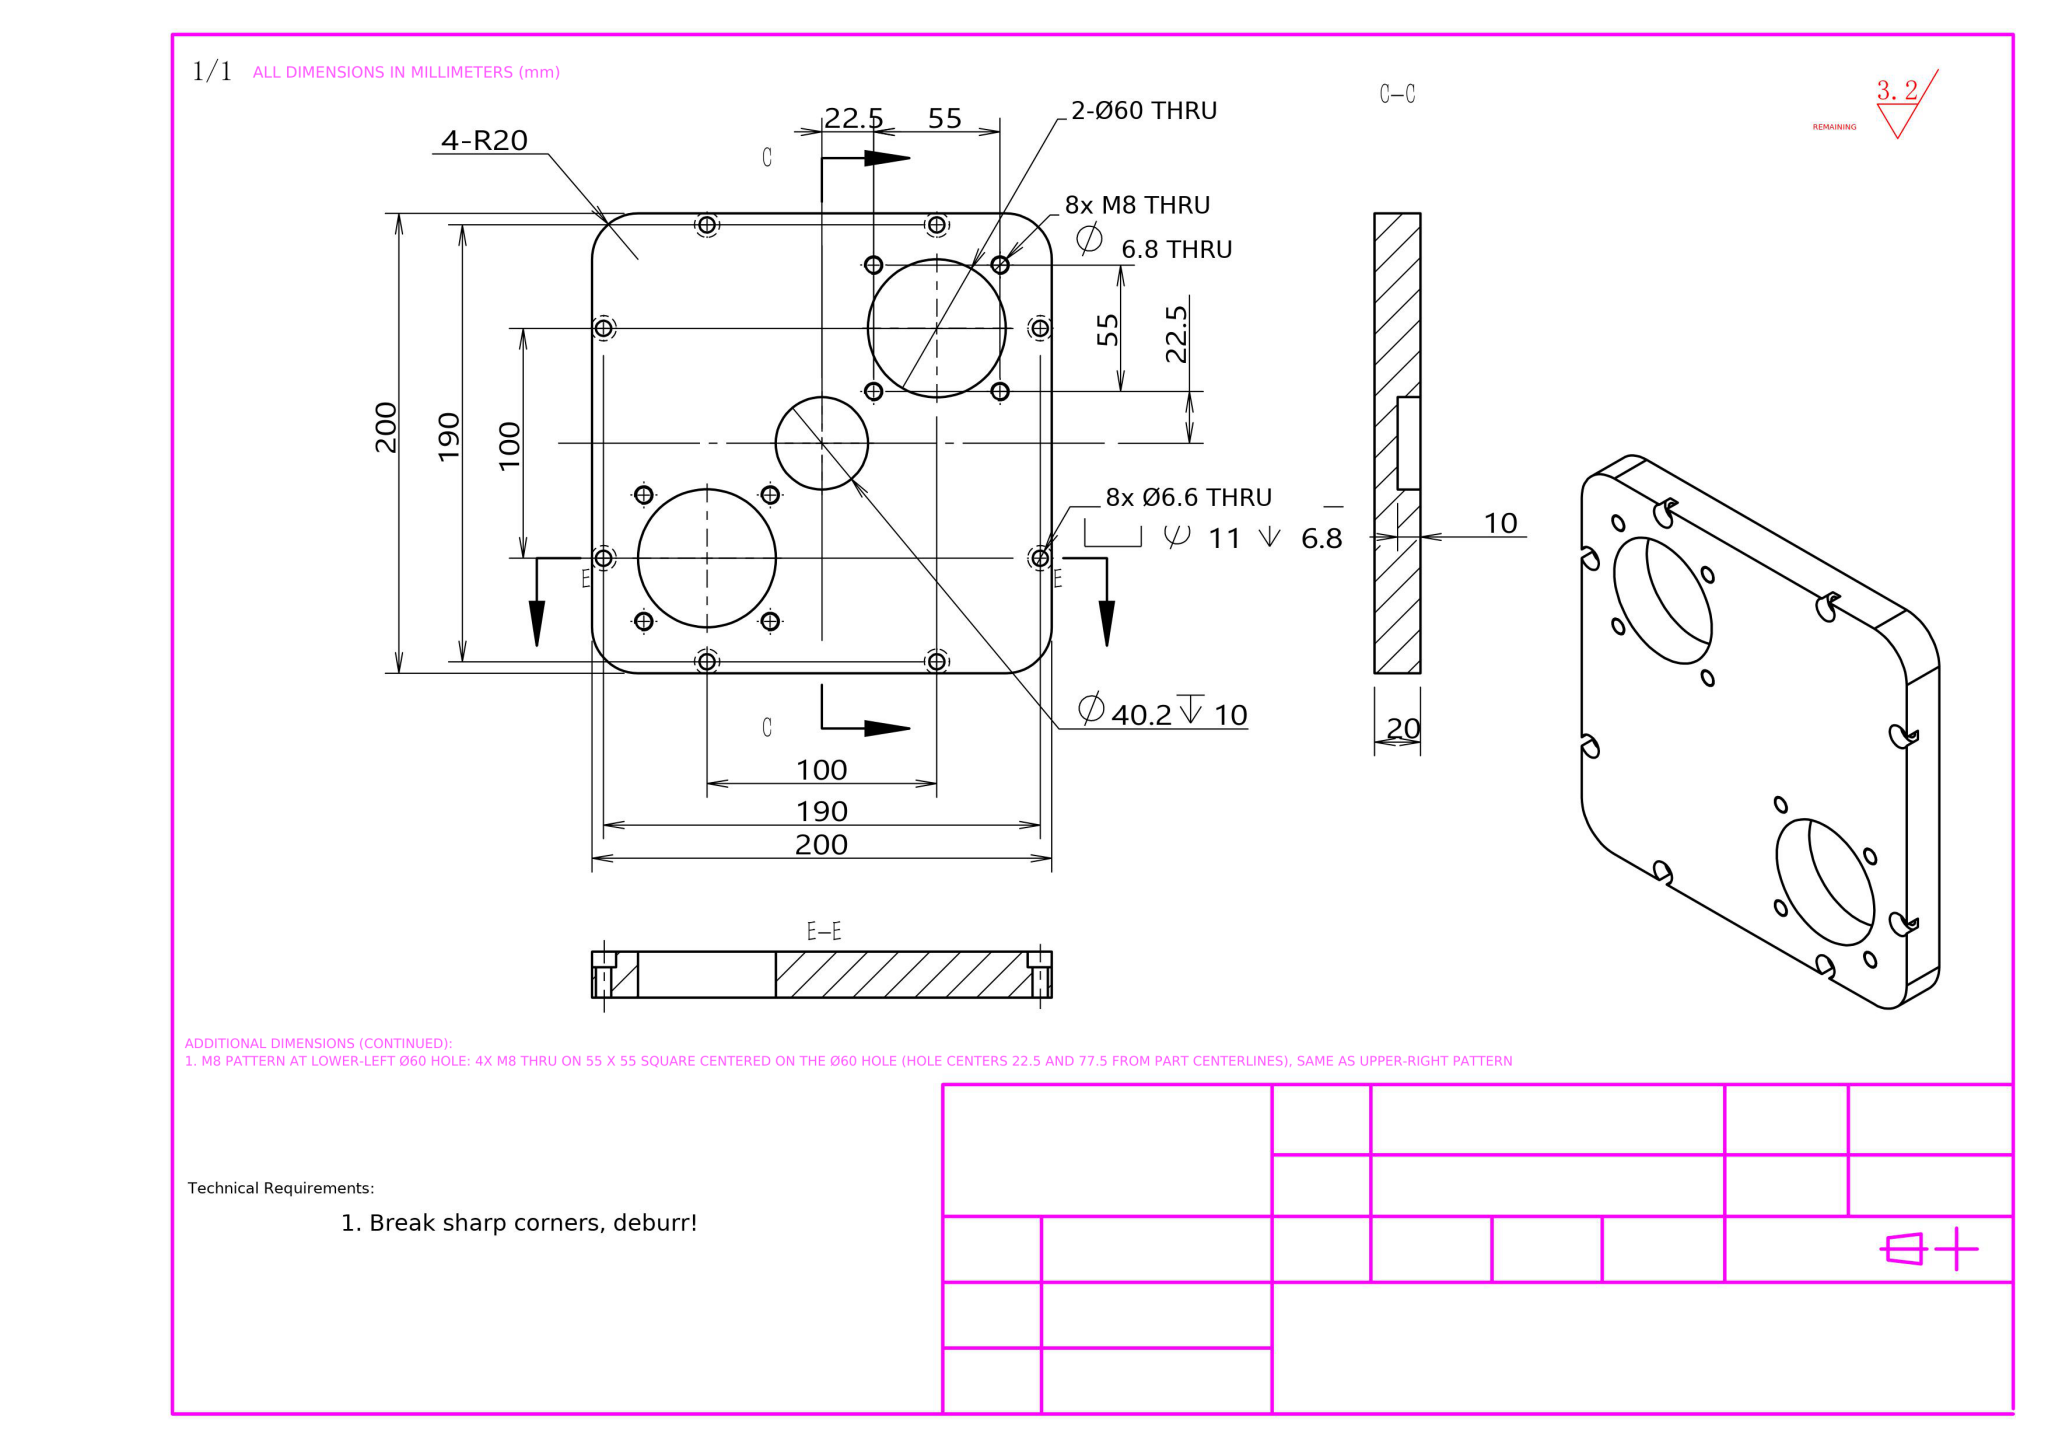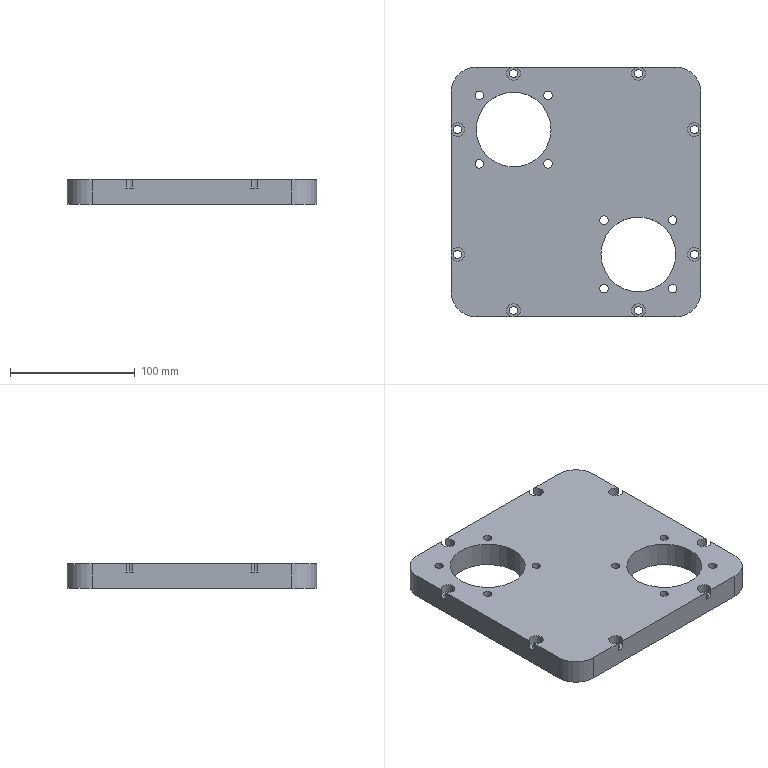Part | NX | mm | 1 solid | 75 faces | box 200 x 200 x 20 mm | volume 652834 mm3 | cylinder 60 | plane 15 | commonest cylinder face diameters 11 x18 6.6 x16 6.8 x16 60 x4 40 x4 40.2 x2